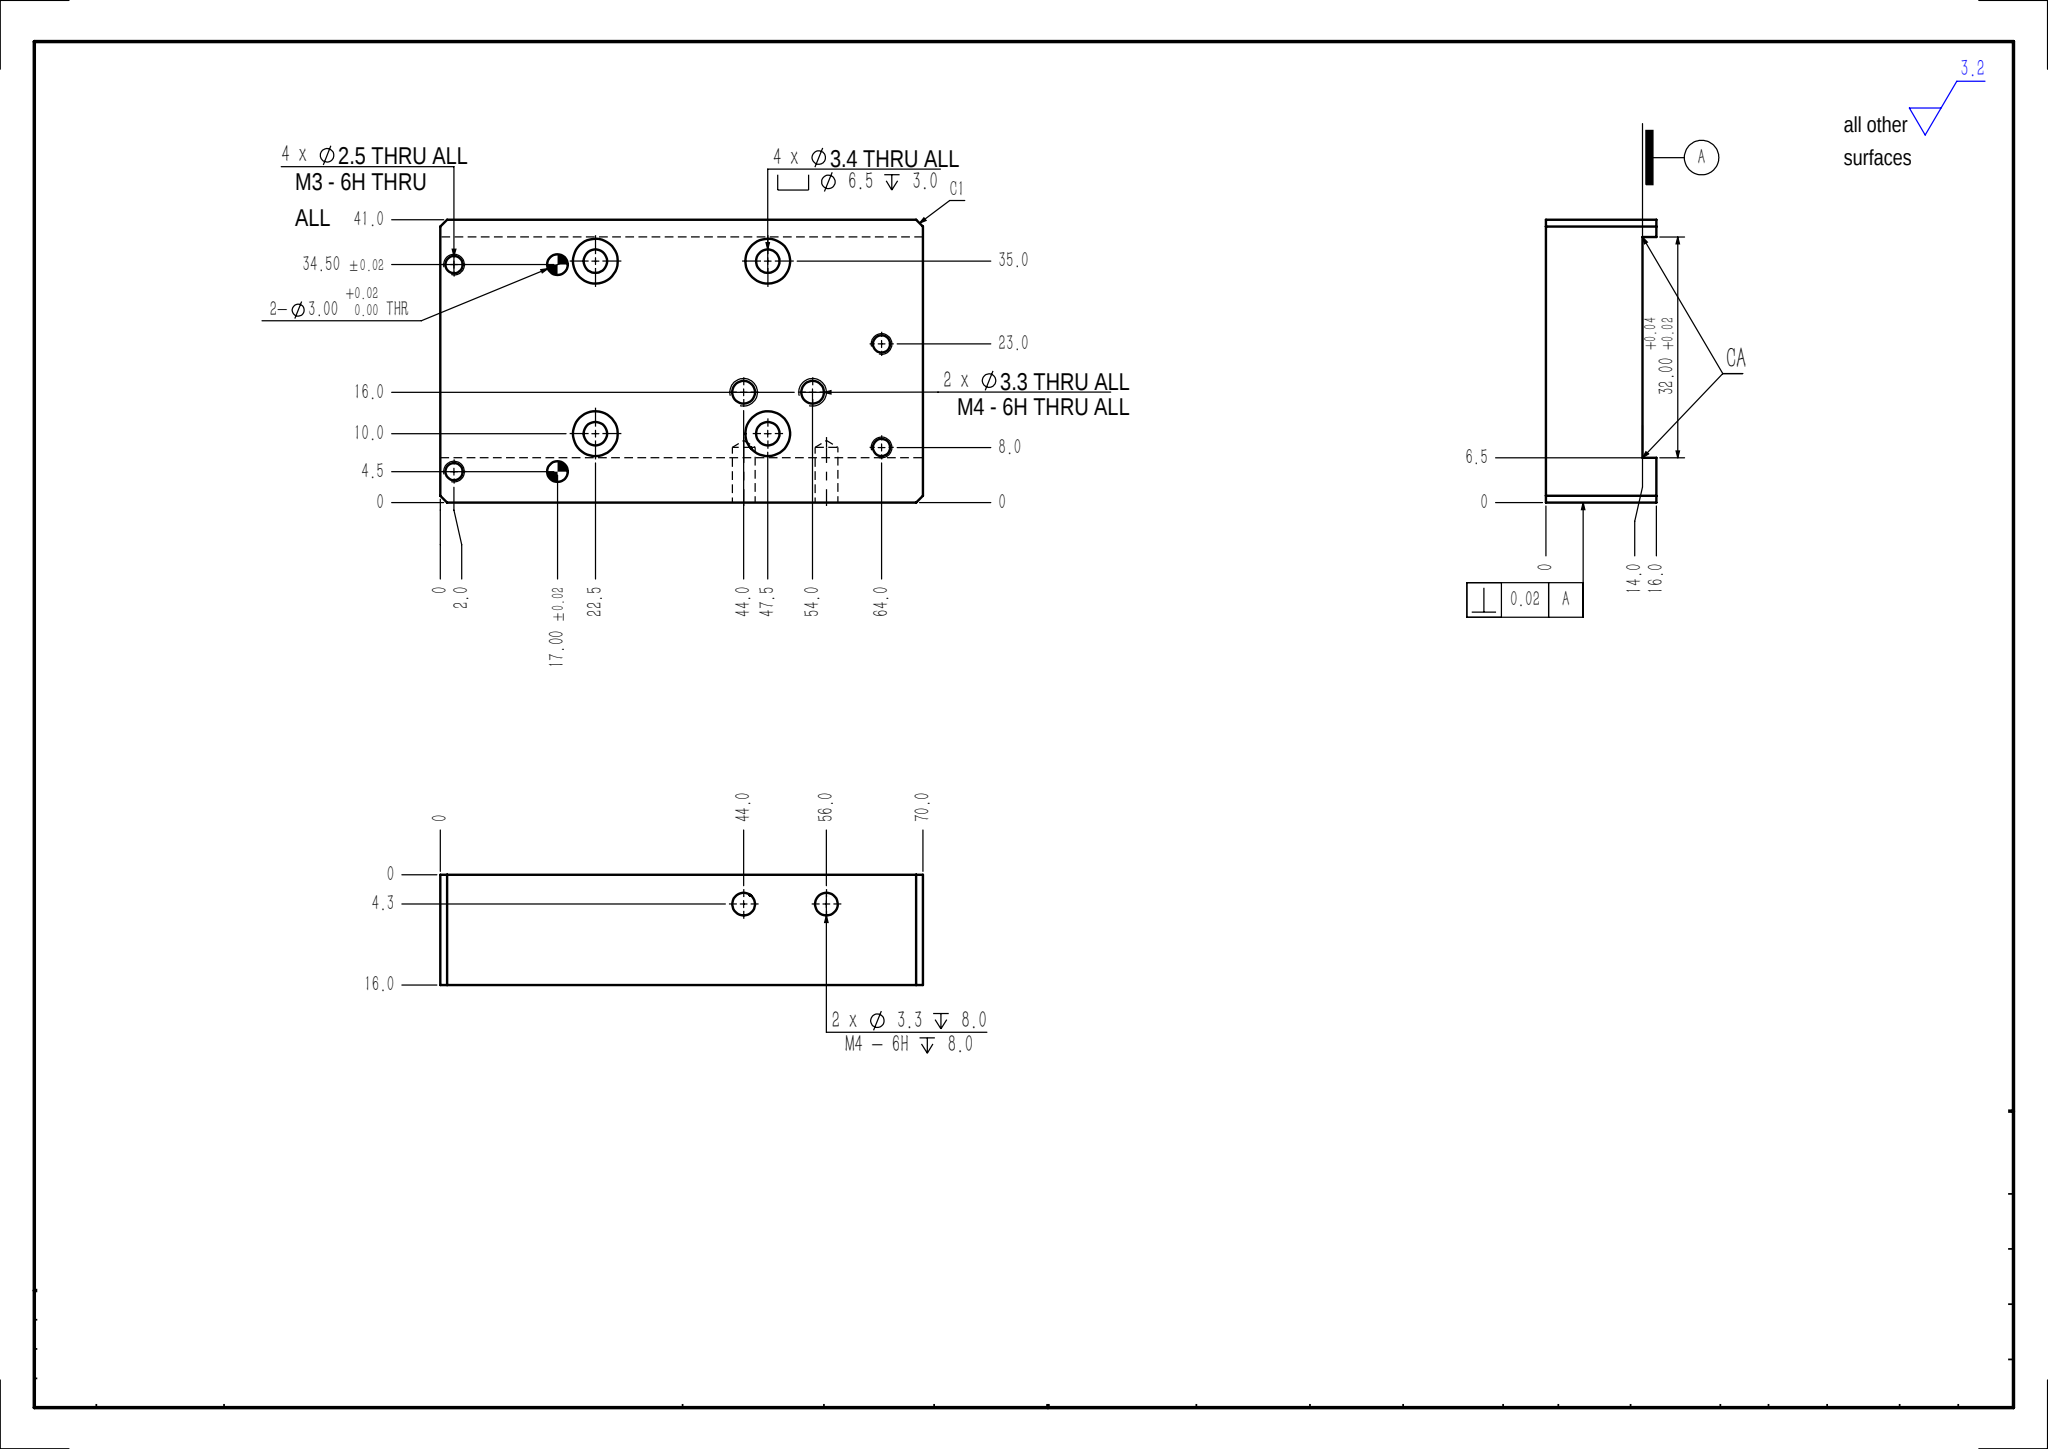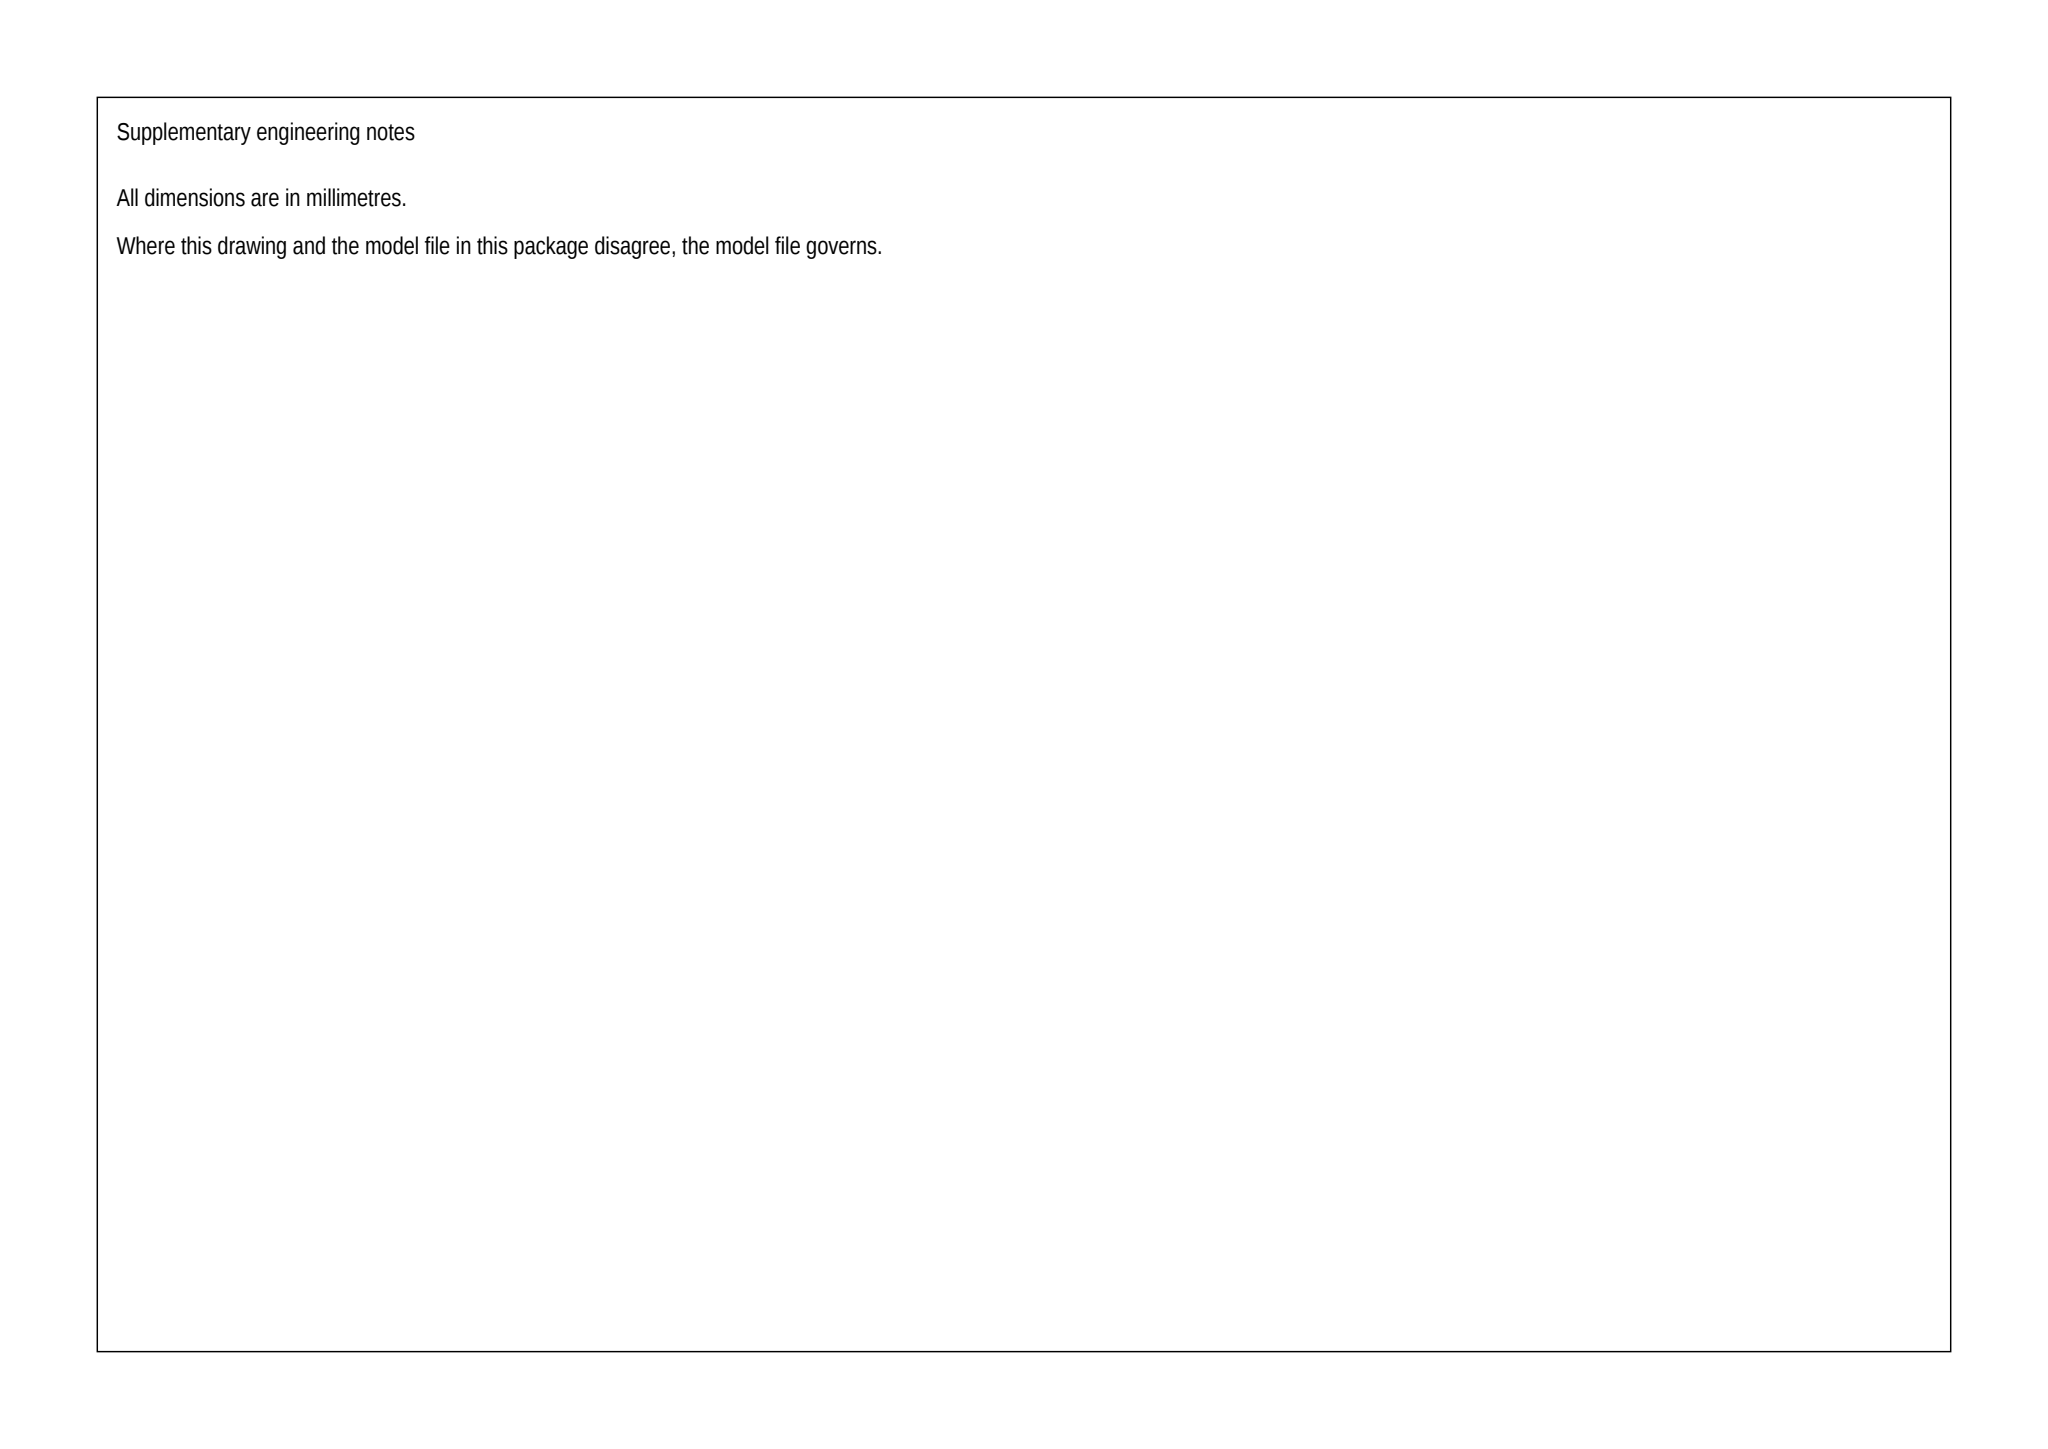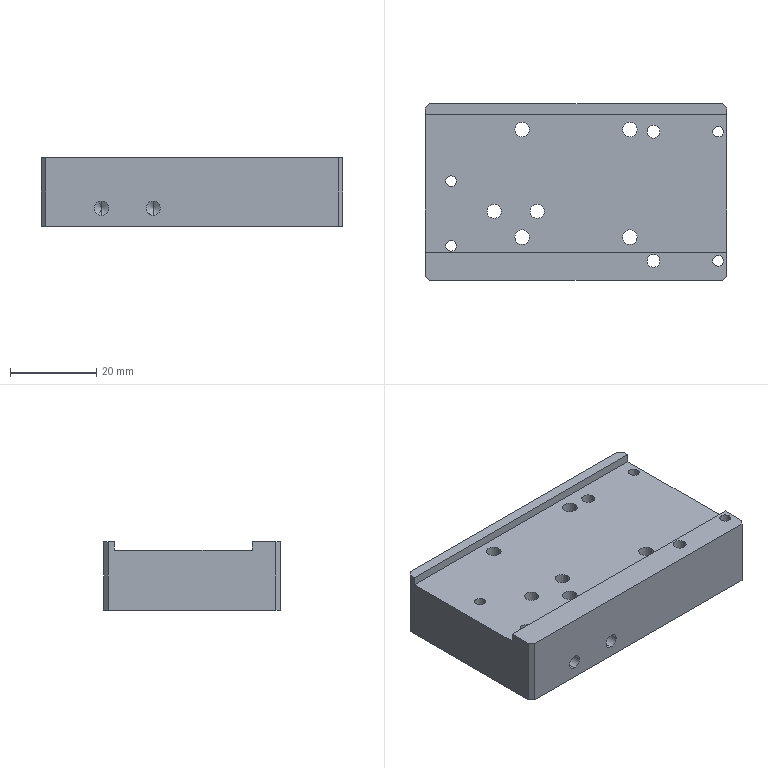Part | SolidWorks | mm | 1 solid | 58 faces | box 70 x 41 x 16 mm | volume 39732 mm3 | cylinder 36 | plane 18 | cone 4 | commonest cylinder face diameters 2.5 x8 3.3 x8 6.5 x8 3.4 x8 3 x4